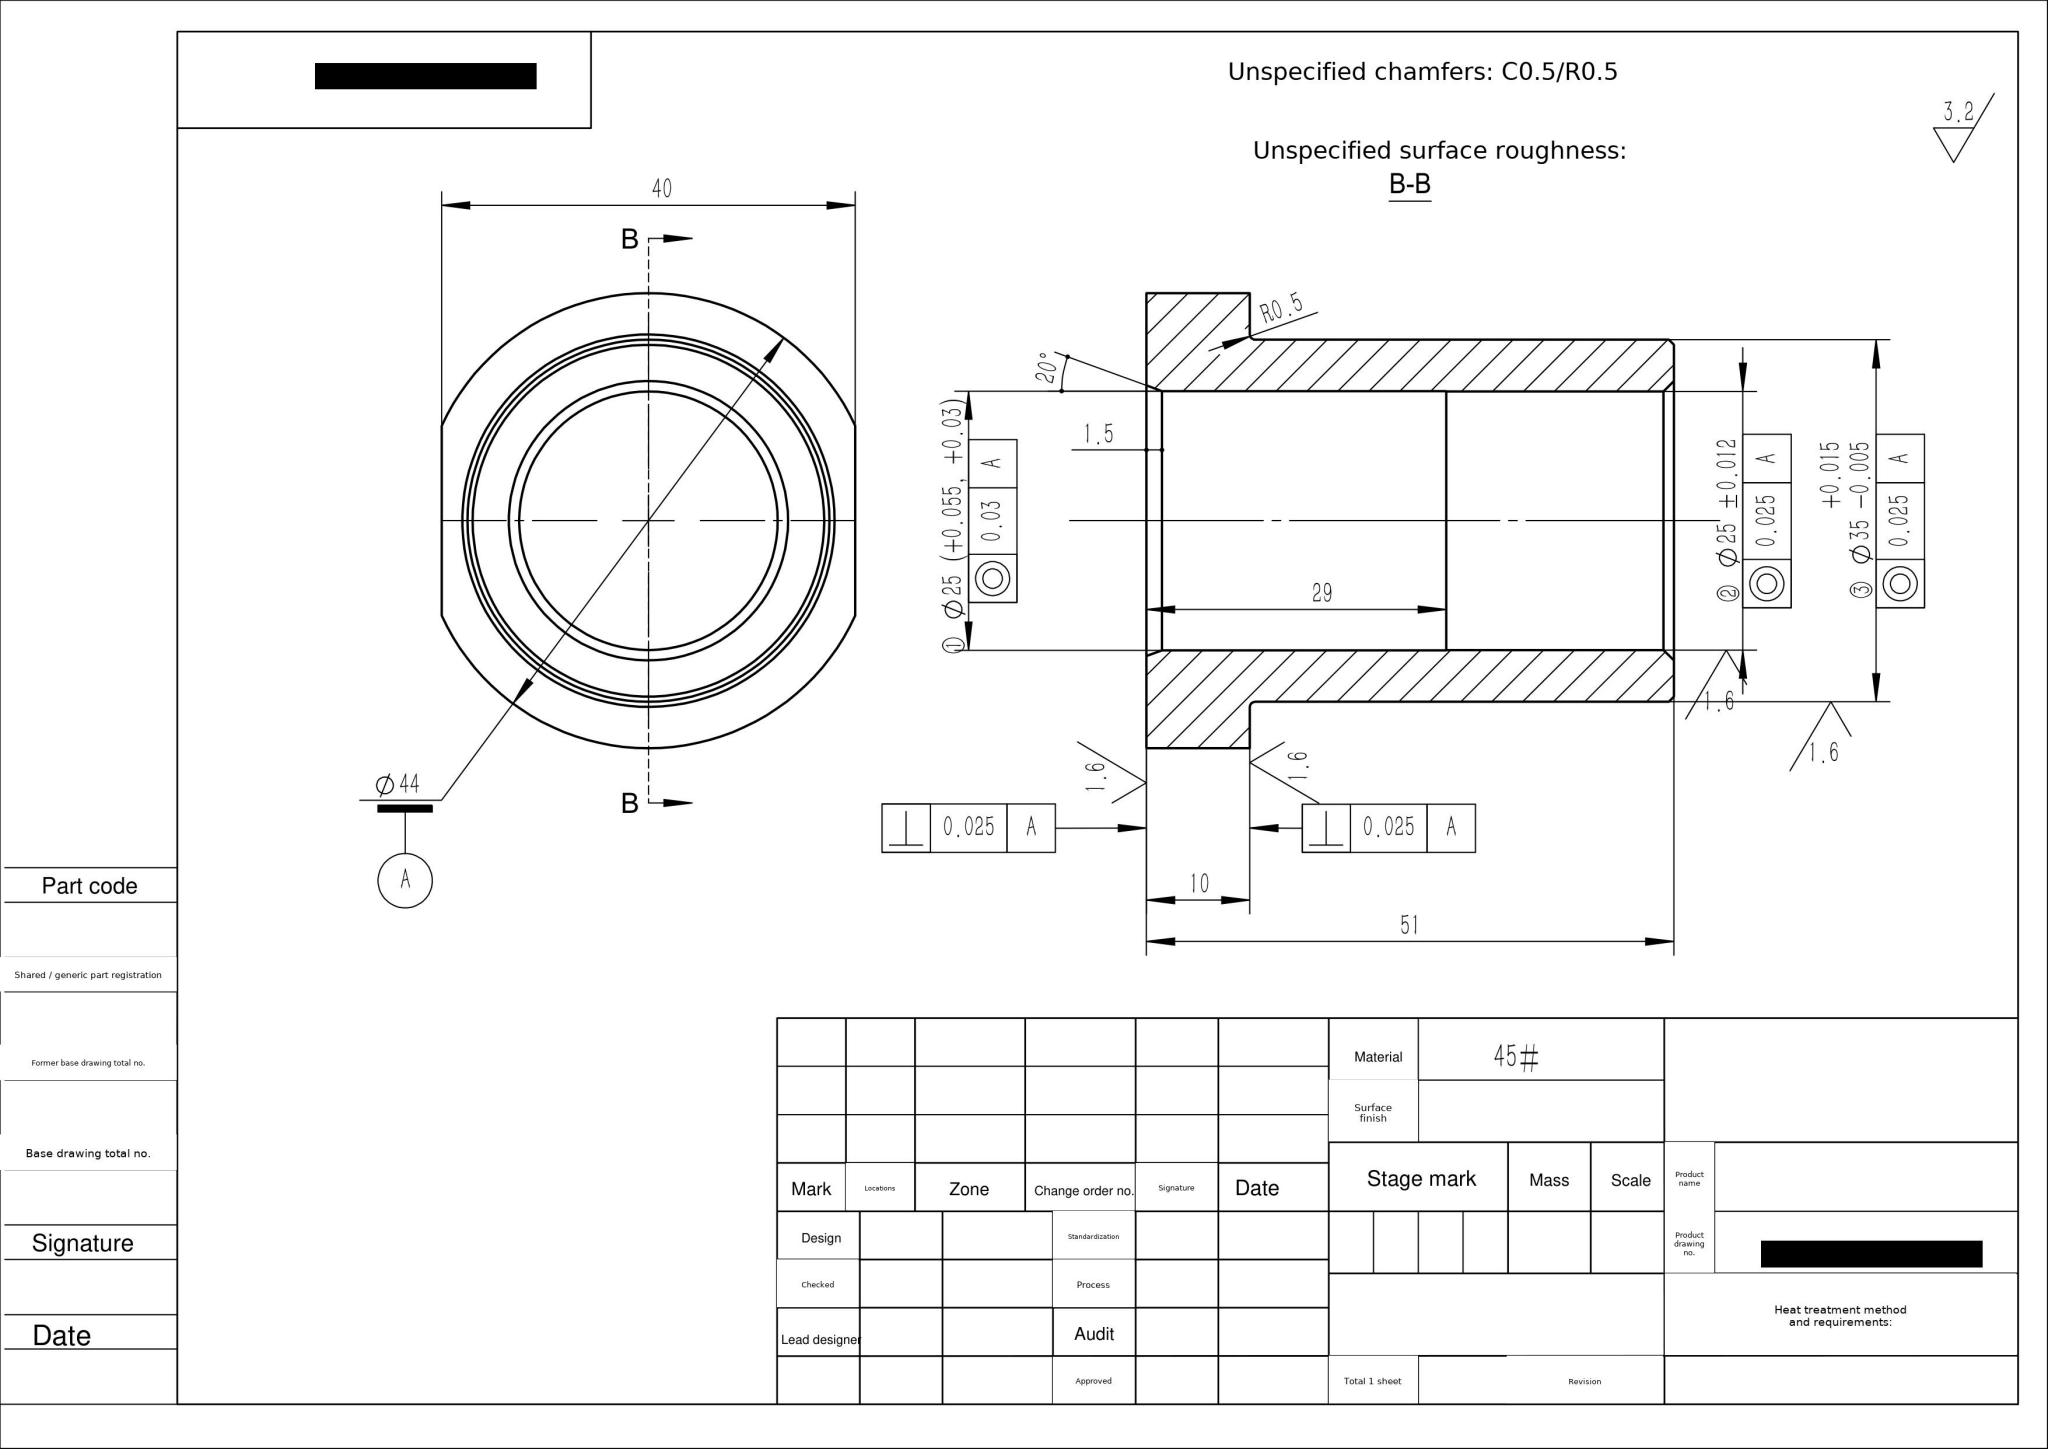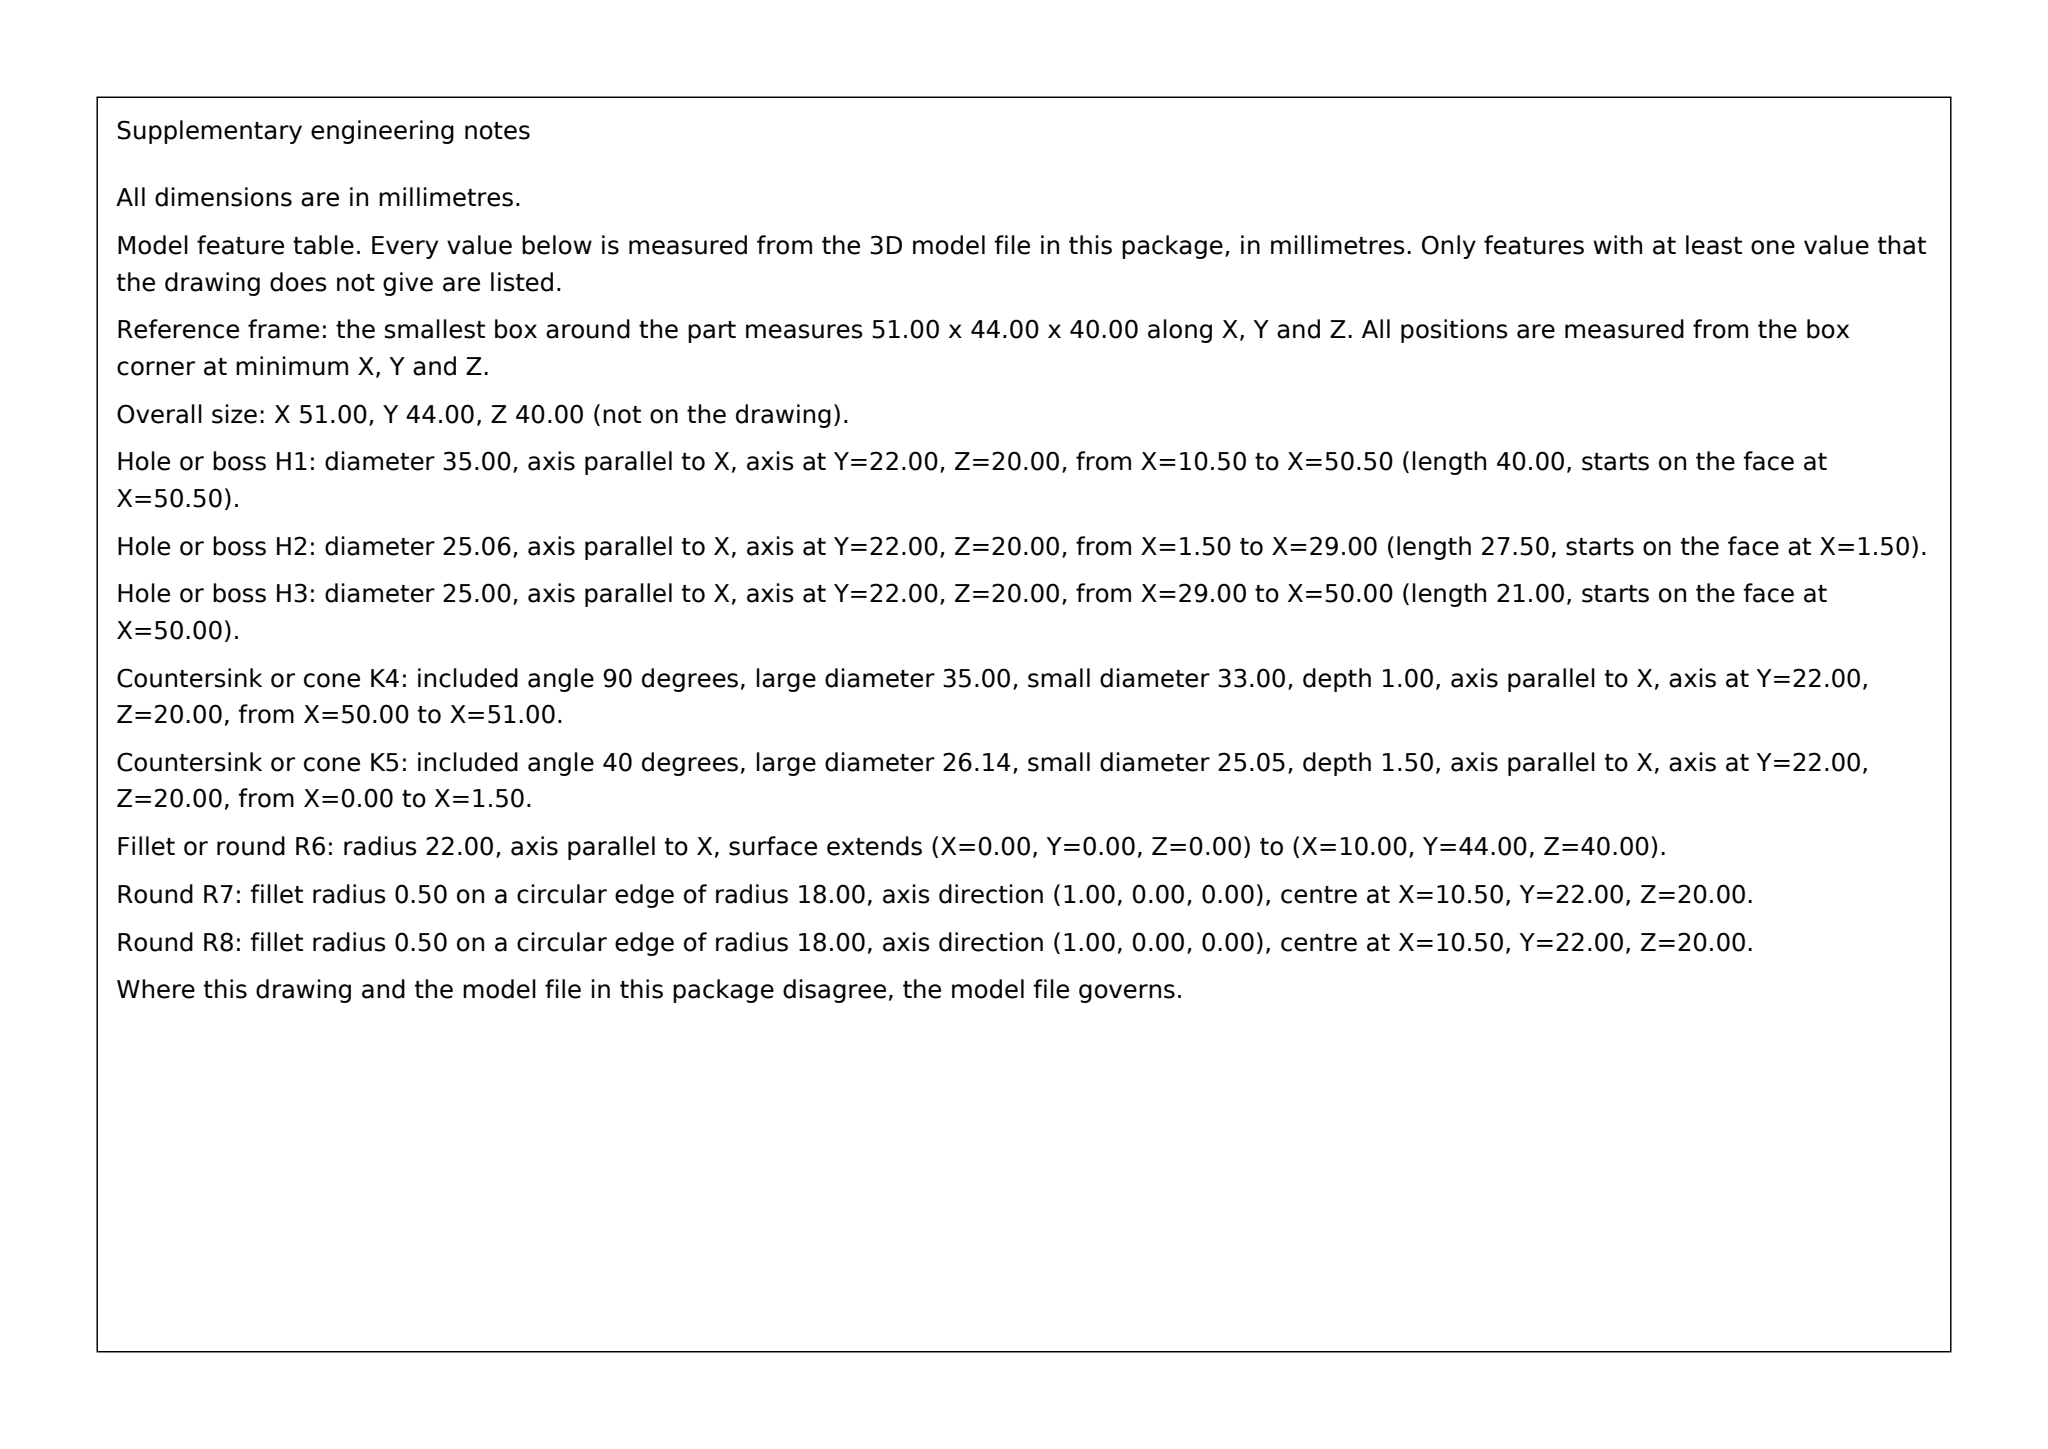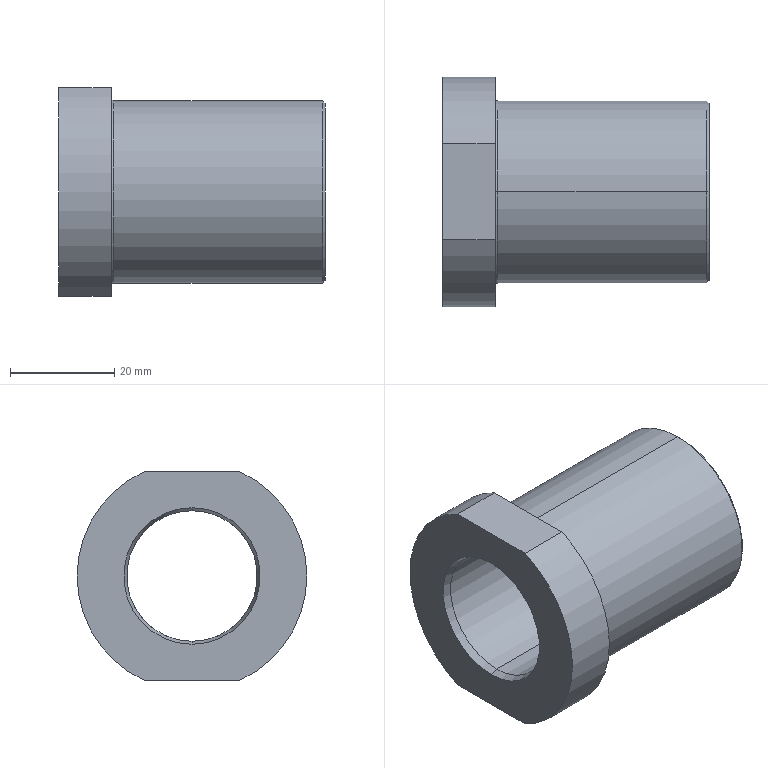Part | SolidWorks | mm | material 45# | 1 solid | 22 faces | box 51 x 44 x 40 mm | volume 28986 mm3 | cylinder 8 | cone 6 | plane 6 | torus 2 | commonest cylinder face diameters 25 x2 35 x2 25.05 x2 44 x2
STEP:
#1=CARTESIAN_POINT('',(50.,0.,12.5));
#2=VERTEX_POINT('',#1);
#3=CARTESIAN_POINT('',(50.,0.,-12.5));
#4=VERTEX_POINT('',#3);
#5=CARTESIAN_POINT('',(50.,0.,0.));
#6=DIRECTION('',(1.,0.,0.));
#7=DIRECTION('',(0.,0.,-1.));
#8=AXIS2_PLACEMENT_3D('',#5,#6,#7);
#9=CIRCLE('',#8,12.5);
#10=EDGE_CURVE('',#2,#4,#9,.T.);
#11=ORIENTED_EDGE('',*,*,#10,.F.);
#12=CARTESIAN_POINT('',(51.,0.,13.5));
#13=VERTEX_POINT('',#12);
#14=CARTESIAN_POINT('',(50.,0.,12.5));
#15=DIRECTION('',(0.7071,0.,0.7071));
#16=VECTOR('',#15,1000.);
#17=LINE('',#14,#16);
#18=EDGE_CURVE('',#2,#13,#17,.T.);
#19=ORIENTED_EDGE('',*,*,#18,.T.);
#20=CARTESIAN_POINT('',(51.,0.,-13.5));
#21=VERTEX_POINT('',#20);
#22=CARTESIAN_POINT('',(51.,0.,0.));
#23=DIRECTION('',(-1.,0.,0.));
#24=DIRECTION('',(0.,0.,-1.));
#25=AXIS2_PLACEMENT_3D('',#22,#23,#24);
#26=CIRCLE('',#25,13.5);
#27=EDGE_CURVE('',#21,#13,#26,.T.);
#28=ORIENTED_EDGE('',*,*,#27,.F.);
#29=CARTESIAN_POINT('',(50.,0.,-12.5));
#30=DIRECTION('',(0.7071,0.,-0.7071));
#31=VECTOR('',#30,1000.);
#32=LINE('',#29,#31);
#33=EDGE_CURVE('',#4,#21,#32,.T.);
#34=ORIENTED_EDGE('',*,*,#33,.F.);
#35=EDGE_LOOP('',(#11,#19,#28,#34));
#36=FACE_OUTER_BOUND('',#35,.T.);
#37=CARTESIAN_POINT('',(50.,0.,0.));
#38=DIRECTION('',(1.,0.,0.));
#39=DIRECTION('',(0.,0.,-1.));
#40=AXIS2_PLACEMENT_3D('',#37,#38,#39);
#41=CONICAL_SURFACE('',#40,12.5,0.7854);
#42=ADVANCED_FACE('',(#36),#41,.F.);
#43=CARTESIAN_POINT('',(29.,0.,12.5));
#44=VERTEX_POINT('',#43);
#45=CARTESIAN_POINT('',(29.,0.,-12.5));
#46=VERTEX_POINT('',#45);
#47=CARTESIAN_POINT('',(29.,0.,0.));
#48=DIRECTION('',(1.,0.,0.));
#49=DIRECTION('',(0.,0.,-1.));
#50=AXIS2_PLACEMENT_3D('',#47,#48,#49);
#51=CIRCLE('',#50,12.5);
#52=EDGE_CURVE('',#44,#46,#51,.T.);
#53=ORIENTED_EDGE('',*,*,#52,.F.);
#54=CARTESIAN_POINT('',(29.,0.,12.5));
#55=DIRECTION('',(1.,0.,0.));
#56=VECTOR('',#55,1000.);
#57=LINE('',#54,#56);
#58=EDGE_CURVE('',#44,#2,#57,.T.);
#59=ORIENTED_EDGE('',*,*,#58,.T.);
#60=ORIENTED_EDGE('',*,*,#10,.T.);
#61=CARTESIAN_POINT('',(29.,0.,-12.5));
#62=DIRECTION('',(1.,0.,0.));
#63=VECTOR('',#62,1000.);
#64=LINE('',#61,#63);
#65=EDGE_CURVE('',#46,#4,#64,.T.);
#66=ORIENTED_EDGE('',*,*,#65,.F.);
#67=EDGE_LOOP('',(#53,#59,#60,#66));
#68=FACE_OUTER_BOUND('',#67,.T.);
#69=CARTESIAN_POINT('',(29.,0.,0.));
#70=DIRECTION('',(1.,0.,0.));
#71=DIRECTION('',(0.,0.,-1.));
#72=AXIS2_PLACEMENT_3D('',#69,#70,#71);
#73=CYLINDRICAL_SURFACE('',#72,12.5);
#74=ADVANCED_FACE('',(#68),#73,.F.);
#75=CARTESIAN_POINT('',(1.5,0.,-12.525));
#76=VERTEX_POINT('',#75);
#77=CARTESIAN_POINT('',(1.5,0.,12.525));
#78=VERTEX_POINT('',#77);
#79=CARTESIAN_POINT('',(1.5,0.,0.));
#80=DIRECTION('',(-1.,0.,0.));
#81=DIRECTION('',(0.,0.,-1.));
#82=AXIS2_PLACEMENT_3D('',#79,#80,#81);
#83=CIRCLE('',#82,12.525);
#84=EDGE_CURVE('',#76,#78,#83,.T.);
#85=ORIENTED_EDGE('',*,*,#84,.F.);
#86=CARTESIAN_POINT('',(0.,0.,-13.071));
#87=VERTEX_POINT('',#86);
#88=CARTESIAN_POINT('',(1.5,0.,-12.525));
#89=DIRECTION('',(-0.9397,0.,-0.342));
#90=VECTOR('',#89,1000.);
#91=LINE('',#88,#90);
#92=EDGE_CURVE('',#76,#87,#91,.T.);
#93=ORIENTED_EDGE('',*,*,#92,.T.);
#94=CARTESIAN_POINT('',(0.,0.,13.071));
#95=VERTEX_POINT('',#94);
#96=CARTESIAN_POINT('',(0.,0.,0.));
#97=DIRECTION('',(1.,0.,0.));
#98=DIRECTION('',(0.,0.,-1.));
#99=AXIS2_PLACEMENT_3D('',#96,#97,#98);
#100=CIRCLE('',#99,13.071);
#101=EDGE_CURVE('',#95,#87,#100,.T.);
#102=ORIENTED_EDGE('',*,*,#101,.F.);
#103=CARTESIAN_POINT('',(1.5,0.,12.525));
#104=DIRECTION('',(-0.9397,0.,0.342));
#105=VECTOR('',#104,1000.);
#106=LINE('',#103,#105);
#107=EDGE_CURVE('',#78,#95,#106,.T.);
#108=ORIENTED_EDGE('',*,*,#107,.F.);
#109=EDGE_LOOP('',(#85,#93,#102,#108));
#110=FACE_OUTER_BOUND('',#109,.T.);
#111=CARTESIAN_POINT('',(1.5,0.,0.));
#112=DIRECTION('',(-1.,0.,0.));
#113=DIRECTION('',(0.,0.,1.));
#114=AXIS2_PLACEMENT_3D('',#111,#112,#113);
#115=CONICAL_SURFACE('',#114,12.525,0.3491);
#116=ADVANCED_FACE('',(#110),#115,.F.);
#117=CARTESIAN_POINT('',(51.,0.,-17.));
#118=VERTEX_POINT('',#117);
#119=CARTESIAN_POINT('',(51.,0.,17.));
#120=VERTEX_POINT('',#119);
#121=CARTESIAN_POINT('',(51.,0.,0.));
#122=DIRECTION('',(1.,0.,0.));
#123=DIRECTION('',(0.,0.,-1.));
#124=AXIS2_PLACEMENT_3D('',#121,#122,#123);
#125=CIRCLE('',#124,17.);
#126=EDGE_CURVE('',#118,#120,#125,.T.);
#127=ORIENTED_EDGE('',*,*,#126,.F.);
#128=CARTESIAN_POINT('',(50.5,0.,-17.5));
#129=VERTEX_POINT('',#128);
#130=CARTESIAN_POINT('',(51.,0.,-17.));
#131=DIRECTION('',(-0.7071,0.,-0.7071));
#132=VECTOR('',#131,1000.);
#133=LINE('',#130,#132);
#134=EDGE_CURVE('',#118,#129,#133,.T.);
#135=ORIENTED_EDGE('',*,*,#134,.T.);
#136=CARTESIAN_POINT('',(50.5,0.,17.5));
#137=VERTEX_POINT('',#136);
#138=CARTESIAN_POINT('',(50.5,0.,0.));
#139=DIRECTION('',(-1.,0.,0.));
#140=DIRECTION('',(0.,0.,-1.));
#141=AXIS2_PLACEMENT_3D('',#138,#139,#140);
#142=CIRCLE('',#141,17.5);
#143=EDGE_CURVE('',#137,#129,#142,.T.);
#144=ORIENTED_EDGE('',*,*,#143,.F.);
#145=CARTESIAN_POINT('',(51.,0.,17.));
#146=DIRECTION('',(-0.7071,0.,0.7071));
#147=VECTOR('',#146,1000.);
#148=LINE('',#145,#147);
#149=EDGE_CURVE('',#120,#137,#148,.T.);
#150=ORIENTED_EDGE('',*,*,#149,.F.);
#151=EDGE_LOOP('',(#127,#135,#144,#150));
#152=FACE_OUTER_BOUND('',#151,.T.);
#153=CARTESIAN_POINT('',(51.,0.,0.));
#154=DIRECTION('',(-1.,0.,0.));
#155=DIRECTION('',(0.,0.,1.));
#156=AXIS2_PLACEMENT_3D('',#153,#154,#155);
#157=CONICAL_SURFACE('',#156,17.,0.7854);
#158=ADVANCED_FACE('',(#152),#157,.T.);
#159=CARTESIAN_POINT('',(10.5,0.,17.5));
#160=VERTEX_POINT('',#159);
#161=CARTESIAN_POINT('',(10.5,0.,-17.5));
#162=VERTEX_POINT('',#161);
#163=CARTESIAN_POINT('',(10.5,0.,0.));
#164=DIRECTION('',(1.,0.,0.));
#165=DIRECTION('',(0.,0.,-1.));
#166=AXIS2_PLACEMENT_3D('',#163,#164,#165);
#167=CIRCLE('',#166,17.5);
#168=EDGE_CURVE('',#160,#162,#167,.T.);
#169=ORIENTED_EDGE('',*,*,#168,.F.);
#170=CARTESIAN_POINT('',(10.,0.,18.));
#171=VERTEX_POINT('',#170);
#172=CARTESIAN_POINT('',(10.5,0.,18.));
#173=DIRECTION('',(0.,1.,-0.));
#174=DIRECTION('',(0.,0.,1.));
#175=AXIS2_PLACEMENT_3D('',#172,#173,#174);
#176=CIRCLE('',#175,0.5);
#177=EDGE_CURVE('',#160,#171,#176,.T.);
#178=ORIENTED_EDGE('',*,*,#177,.T.);
#179=CARTESIAN_POINT('',(10.,0.,-18.));
#180=VERTEX_POINT('',#179);
#181=CARTESIAN_POINT('',(10.,0.,0.));
#182=DIRECTION('',(-1.,0.,0.));
#183=DIRECTION('',(0.,0.,-1.));
#184=AXIS2_PLACEMENT_3D('',#181,#182,#183);
#185=CIRCLE('',#184,18.);
#186=EDGE_CURVE('',#180,#171,#185,.T.);
#187=ORIENTED_EDGE('',*,*,#186,.F.);
#188=CARTESIAN_POINT('',(10.5,0.,-18.));
#189=DIRECTION('',(0.,-1.,0.));
#190=DIRECTION('',(0.,0.,-1.));
#191=AXIS2_PLACEMENT_3D('',#188,#189,#190);
#192=CIRCLE('',#191,0.5);
#193=EDGE_CURVE('',#162,#180,#192,.T.);
#194=ORIENTED_EDGE('',*,*,#193,.F.);
#195=EDGE_LOOP('',(#169,#178,#187,#194));
#196=FACE_OUTER_BOUND('',#195,.T.);
#197=CARTESIAN_POINT('',(10.5,0.,0.));
#198=DIRECTION('',(1.,0.,0.));
#199=DIRECTION('',(0.,0.,-1.));
#200=AXIS2_PLACEMENT_3D('',#197,#198,#199);
#201=TOROIDAL_SURFACE('',#200,18.,0.5);
#202=ADVANCED_FACE('',(#196),#201,.F.);
#203=ORIENTED_EDGE('',*,*,#143,.T.);
#204=CARTESIAN_POINT('',(51.,0.,-17.5));
#205=DIRECTION('',(-1.,0.,0.));
#206=VECTOR('',#205,1000.);
#207=LINE('',#204,#206);
#208=EDGE_CURVE('',#129,#162,#207,.T.);
#209=ORIENTED_EDGE('',*,*,#208,.T.);
#210=CARTESIAN_POINT('',(10.5,0.,0.));
#211=DIRECTION('',(1.,0.,0.));
#212=DIRECTION('',(0.,0.,-1.));
#213=AXIS2_PLACEMENT_3D('',#210,#211,#212);
#214=CIRCLE('',#213,17.5);
#215=EDGE_CURVE('',#162,#160,#214,.T.);
#216=ORIENTED_EDGE('',*,*,#215,.T.);
#217=CARTESIAN_POINT('',(51.,0.,17.5));
#218=DIRECTION('',(-1.,0.,0.));
#219=VECTOR('',#218,1000.);
#220=LINE('',#217,#219);
#221=EDGE_CURVE('',#137,#160,#220,.T.);
#222=ORIENTED_EDGE('',*,*,#221,.F.);
#223=EDGE_LOOP('',(#203,#209,#216,#222));
#224=FACE_OUTER_BOUND('',#223,.T.);
#225=CARTESIAN_POINT('',(51.,0.,0.));
#226=DIRECTION('',(-1.,0.,0.));
#227=DIRECTION('',(0.,0.,1.));
#228=AXIS2_PLACEMENT_3D('',#225,#226,#227);
#229=CYLINDRICAL_SURFACE('',#228,17.5);
#230=ADVANCED_FACE('',(#224),#229,.T.);
#231=CARTESIAN_POINT('',(29.,0.,-12.525));
#232=VERTEX_POINT('',#231);
#233=CARTESIAN_POINT('',(29.,0.,12.525));
#234=VERTEX_POINT('',#233);
#235=CARTESIAN_POINT('',(29.,0.,0.));
#236=DIRECTION('',(-1.,0.,0.));
#237=DIRECTION('',(0.,0.,-1.));
#238=AXIS2_PLACEMENT_3D('',#235,#236,#237);
#239=CIRCLE('',#238,12.525);
#240=EDGE_CURVE('',#232,#234,#239,.T.);
#241=ORIENTED_EDGE('',*,*,#240,.F.);
#242=CARTESIAN_POINT('',(51.,0.,-12.525));
#243=DIRECTION('',(-1.,0.,0.));
#244=VECTOR('',#243,1000.);
#245=LINE('',#242,#244);
#246=EDGE_CURVE('',#232,#76,#245,.T.);
#247=ORIENTED_EDGE('',*,*,#246,.T.);
#248=ORIENTED_EDGE('',*,*,#84,.T.);
#249=CARTESIAN_POINT('',(51.,0.,12.525));
#250=DIRECTION('',(-1.,0.,0.));
#251=VECTOR('',#250,1000.);
#252=LINE('',#249,#251);
#253=EDGE_CURVE('',#234,#78,#252,.T.);
#254=ORIENTED_EDGE('',*,*,#253,.F.);
#255=EDGE_LOOP('',(#241,#247,#248,#254));
#256=FACE_OUTER_BOUND('',#255,.T.);
#257=CARTESIAN_POINT('',(51.,0.,0.));
#258=DIRECTION('',(-1.,0.,0.));
#259=DIRECTION('',(0.,0.,1.));
#260=AXIS2_PLACEMENT_3D('',#257,#258,#259);
#261=CYLINDRICAL_SURFACE('',#260,12.525);
#262=ADVANCED_FACE('',(#256),#261,.F.);
#263=ORIENTED_EDGE('',*,*,#246,.F.);
#264=CARTESIAN_POINT('',(29.,0.,0.));
#265=DIRECTION('',(-1.,0.,0.));
#266=DIRECTION('',(0.,0.,-1.));
#267=AXIS2_PLACEMENT_3D('',#264,#265,#266);
#268=CIRCLE('',#267,12.525);
#269=EDGE_CURVE('',#234,#232,#268,.T.);
#270=ORIENTED_EDGE('',*,*,#269,.F.);
#271=ORIENTED_EDGE('',*,*,#253,.T.);
#272=CARTESIAN_POINT('',(1.5,0.,0.));
#273=DIRECTION('',(-1.,0.,0.));
#274=DIRECTION('',(0.,0.,-1.));
#275=AXIS2_PLACEMENT_3D('',#272,#273,#274);
#276=CIRCLE('',#275,12.525);
#277=EDGE_CURVE('',#78,#76,#276,.T.);
#278=ORIENTED_EDGE('',*,*,#277,.T.);
#279=EDGE_LOOP('',(#263,#270,#271,#278));
#280=FACE_OUTER_BOUND('',#279,.T.);
#281=CARTESIAN_POINT('',(51.,0.,0.));
#282=DIRECTION('',(-1.,0.,0.));
#283=DIRECTION('',(0.,0.,1.));
#284=AXIS2_PLACEMENT_3D('',#281,#282,#283);
#285=CYLINDRICAL_SURFACE('',#284,12.525);
#286=ADVANCED_FACE('',(#280),#285,.F.);
#287=CARTESIAN_POINT('',(10.,9.165,20.));
#288=VERTEX_POINT('',#287);
#289=CARTESIAN_POINT('',(0.,9.165,20.));
#290=VERTEX_POINT('',#289);
#291=CARTESIAN_POINT('',(10.,9.165,20.));
#292=DIRECTION('',(-1.,0.,0.));
#293=VECTOR('',#292,1000.);
#294=LINE('',#291,#293);
#295=EDGE_CURVE('',#288,#290,#294,.T.);
#296=ORIENTED_EDGE('',*,*,#295,.F.);
#297=CARTESIAN_POINT('',(10.,9.165,-20.));
#298=VERTEX_POINT('',#297);
#299=CARTESIAN_POINT('',(10.,0.,0.));
#300=DIRECTION('',(1.,0.,0.));
#301=DIRECTION('',(0.,0.,-1.));
#302=AXIS2_PLACEMENT_3D('',#299,#300,#301);
#303=CIRCLE('',#302,22.);
#304=EDGE_CURVE('',#298,#288,#303,.T.);
#305=ORIENTED_EDGE('',*,*,#304,.F.);
#306=CARTESIAN_POINT('',(0.,9.165,-20.));
#307=VERTEX_POINT('',#306);
#308=CARTESIAN_POINT('',(10.,9.165,-20.));
#309=DIRECTION('',(1.,0.,0.));
#310=VECTOR('',#309,1000.);
#311=LINE('',#308,#310);
#312=EDGE_CURVE('',#307,#298,#311,.T.);
#313=ORIENTED_EDGE('',*,*,#312,.F.);
#314=CARTESIAN_POINT('',(0.,0.,0.));
#315=DIRECTION('',(1.,0.,0.));
#316=DIRECTION('',(0.,0.,-1.));
#317=AXIS2_PLACEMENT_3D('',#314,#315,#316);
#318=CIRCLE('',#317,22.);
#319=EDGE_CURVE('',#307,#290,#318,.T.);
#320=ORIENTED_EDGE('',*,*,#319,.T.);
#321=EDGE_LOOP('',(#296,#305,#313,#320));
#322=FACE_OUTER_BOUND('',#321,.T.);
#323=CARTESIAN_POINT('',(10.,0.,0.));
#324=DIRECTION('',(-1.,0.,0.));
#325=DIRECTION('',(0.,0.,1.));
#326=AXIS2_PLACEMENT_3D('',#323,#324,#325);
#327=CYLINDRICAL_SURFACE('',#326,22.);
#328=ADVANCED_FACE('',(#322),#327,.T.);
#329=CARTESIAN_POINT('',(0.,-9.165,20.));
#330=VERTEX_POINT('',#329);
#331=CARTESIAN_POINT('',(10.,-9.165,20.));
#332=VERTEX_POINT('',#331);
#333=CARTESIAN_POINT('',(10.,-9.165,20.));
#334=DIRECTION('',(1.,0.,0.));
#335=VECTOR('',#334,1000.);
#336=LINE('',#333,#335);
#337=EDGE_CURVE('',#330,#332,#336,.T.);
#338=ORIENTED_EDGE('',*,*,#337,.F.);
#339=CARTESIAN_POINT('',(0.,-9.165,-20.));
#340=VERTEX_POINT('',#339);
#341=CARTESIAN_POINT('',(0.,0.,0.));
#342=DIRECTION('',(1.,0.,0.));
#343=DIRECTION('',(0.,0.,-1.));
#344=AXIS2_PLACEMENT_3D('',#341,#342,#343);
#345=CIRCLE('',#344,22.);
#346=EDGE_CURVE('',#330,#340,#345,.T.);
#347=ORIENTED_EDGE('',*,*,#346,.T.);
#348=CARTESIAN_POINT('',(10.,-9.165,-20.));
#349=VERTEX_POINT('',#348);
#350=CARTESIAN_POINT('',(10.,-9.165,-20.));
#351=DIRECTION('',(-1.,0.,0.));
#352=VECTOR('',#351,1000.);
#353=LINE('',#350,#352);
#354=EDGE_CURVE('',#349,#340,#353,.T.);
#355=ORIENTED_EDGE('',*,*,#354,.F.);
#356=CARTESIAN_POINT('',(10.,0.,0.));
#357=DIRECTION('',(1.,0.,0.));
#358=DIRECTION('',(0.,0.,-1.));
#359=AXIS2_PLACEMENT_3D('',#356,#357,#358);
#360=CIRCLE('',#359,22.);
#361=EDGE_CURVE('',#332,#349,#360,.T.);
#362=ORIENTED_EDGE('',*,*,#361,.F.);
#363=EDGE_LOOP('',(#338,#347,#355,#362));
#364=FACE_OUTER_BOUND('',#363,.T.);
#365=CARTESIAN_POINT('',(10.,0.,0.));
#366=DIRECTION('',(-1.,0.,0.));
#367=DIRECTION('',(0.,0.,1.));
#368=AXIS2_PLACEMENT_3D('',#365,#366,#367);
#369=CYLINDRICAL_SURFACE('',#368,22.);
#370=ADVANCED_FACE('',(#364),#369,.T.);
#371=ORIENTED_EDGE('',*,*,#186,.T.);
#372=CARTESIAN_POINT('',(10.,0.,0.));
#373=DIRECTION('',(-1.,0.,0.));
#374=DIRECTION('',(0.,0.,-1.));
#375=AXIS2_PLACEMENT_3D('',#372,#373,#374);
#376=CIRCLE('',#375,18.);
#377=EDGE_CURVE('',#171,#180,#376,.T.);
#378=ORIENTED_EDGE('',*,*,#377,.T.);
#379=EDGE_LOOP('',(#371,#378));
#380=FACE_BOUND('',#379,.T.);
#381=ORIENTED_EDGE('',*,*,#304,.T.);
#382=CARTESIAN_POINT('',(10.,0.,20.));
#383=DIRECTION('',(0.,-1.,0.));
#384=VECTOR('',#383,1000.);
#385=LINE('',#382,#384);
#386=EDGE_CURVE('',#288,#332,#385,.T.);
#387=ORIENTED_EDGE('',*,*,#386,.T.);
#388=ORIENTED_EDGE('',*,*,#361,.T.);
#389=CARTESIAN_POINT('',(10.,-0.,-20.));
#390=DIRECTION('',(0.,1.,-0.));
#391=VECTOR('',#390,1000.);
#392=LINE('',#389,#391);
#393=EDGE_CURVE('',#349,#298,#392,.T.);
#394=ORIENTED_EDGE('',*,*,#393,.T.);
#395=EDGE_LOOP('',(#381,#387,#388,#394));
#396=FACE_OUTER_BOUND('',#395,.T.);
#397=CARTESIAN_POINT('',(10.,0.,0.));
#398=DIRECTION('',(1.,0.,0.));
#399=DIRECTION('',(0.,0.,-1.));
#400=AXIS2_PLACEMENT_3D('',#397,#398,#399);
#401=PLANE('',#400);
#402=ADVANCED_FACE('',(#380,#396),#401,.T.);
#403=ORIENTED_EDGE('',*,*,#101,.T.);
#404=CARTESIAN_POINT('',(0.,0.,0.));
#405=DIRECTION('',(1.,0.,0.));
#406=DIRECTION('',(0.,0.,-1.));
#407=AXIS2_PLACEMENT_3D('',#404,#405,#406);
#408=CIRCLE('',#407,13.071);
#409=EDGE_CURVE('',#87,#95,#408,.T.);
#410=ORIENTED_EDGE('',*,*,#409,.T.);
#411=EDGE_LOOP('',(#403,#410));
#412=FACE_BOUND('',#411,.T.);
#413=CARTESIAN_POINT('',(0.,0.,20.));
#414=DIRECTION('',(0.,-1.,0.));
#415=VECTOR('',#414,1000.);
#416=LINE('',#413,#415);
#417=EDGE_CURVE('',#290,#330,#416,.T.);
#418=ORIENTED_EDGE('',*,*,#417,.F.);
#419=ORIENTED_EDGE('',*,*,#319,.F.);
#420=CARTESIAN_POINT('',(0.,-0.,-20.));
#421=DIRECTION('',(0.,1.,-0.));
#422=VECTOR('',#421,1000.);
#423=LINE('',#420,#422);
#424=EDGE_CURVE('',#340,#307,#423,.T.);
#425=ORIENTED_EDGE('',*,*,#424,.F.);
#426=ORIENTED_EDGE('',*,*,#346,.F.);
#427=EDGE_LOOP('',(#418,#419,#425,#426));
#428=FACE_OUTER_BOUND('',#427,.T.);
#429=CARTESIAN_POINT('',(0.,0.,0.));
#430=DIRECTION('',(1.,0.,0.));
#431=DIRECTION('',(0.,0.,-1.));
#432=AXIS2_PLACEMENT_3D('',#429,#430,#431);
#433=PLANE('',#432);
#434=ADVANCED_FACE('',(#412,#428),#433,.F.);
#435=ORIENTED_EDGE('',*,*,#208,.F.);
#436=CARTESIAN_POINT('',(50.5,0.,0.));
#437=DIRECTION('',(-1.,0.,0.));
#438=DIRECTION('',(0.,0.,-1.));
#439=AXIS2_PLACEMENT_3D('',#436,#437,#438);
#440=CIRCLE('',#439,17.5);
#441=EDGE_CURVE('',#129,#137,#440,.T.);
#442=ORIENTED_EDGE('',*,*,#441,.T.);
#443=ORIENTED_EDGE('',*,*,#221,.T.);
#444=ORIENTED_EDGE('',*,*,#168,.T.);
#445=EDGE_LOOP('',(#435,#442,#443,#444));
#446=FACE_OUTER_BOUND('',#445,.T.);
#447=CARTESIAN_POINT('',(51.,0.,0.));
#448=DIRECTION('',(-1.,0.,0.));
#449=DIRECTION('',(0.,0.,1.));
#450=AXIS2_PLACEMENT_3D('',#447,#448,#449);
#451=CYLINDRICAL_SURFACE('',#450,17.5);
#452=ADVANCED_FACE('',(#446),#451,.T.);
#453=ORIENTED_EDGE('',*,*,#27,.T.);
#454=CARTESIAN_POINT('',(51.,0.,0.));
#455=DIRECTION('',(-1.,0.,0.));
#456=DIRECTION('',(0.,0.,-1.));
#457=AXIS2_PLACEMENT_3D('',#454,#455,#456);
#458=CIRCLE('',#457,13.5);
#459=EDGE_CURVE('',#13,#21,#458,.T.);
#460=ORIENTED_EDGE('',*,*,#459,.T.);
#461=EDGE_LOOP('',(#453,#460));
#462=FACE_BOUND('',#461,.T.);
#463=CARTESIAN_POINT('',(51.,0.,0.));
#464=DIRECTION('',(1.,0.,0.));
#465=DIRECTION('',(0.,0.,-1.));
#466=AXIS2_PLACEMENT_3D('',#463,#464,#465);
#467=CIRCLE('',#466,17.);
#468=EDGE_CURVE('',#120,#118,#467,.T.);
#469=ORIENTED_EDGE('',*,*,#468,.T.);
#470=ORIENTED_EDGE('',*,*,#126,.T.);
#471=EDGE_LOOP('',(#469,#470));
#472=FACE_OUTER_BOUND('',#471,.T.);
#473=CARTESIAN_POINT('',(51.,0.,0.));
#474=DIRECTION('',(1.,0.,0.));
#475=DIRECTION('',(0.,0.,-1.));
#476=AXIS2_PLACEMENT_3D('',#473,#474,#475);
#477=PLANE('',#476);
#478=ADVANCED_FACE('',(#462,#472),#477,.T.);
#479=ORIENTED_EDGE('',*,*,#354,.T.);
#480=ORIENTED_EDGE('',*,*,#424,.T.);
#481=ORIENTED_EDGE('',*,*,#312,.T.);
#482=ORIENTED_EDGE('',*,*,#393,.F.);
#483=EDGE_LOOP('',(#479,#480,#481,#482));
#484=FACE_OUTER_BOUND('',#483,.T.);
#485=CARTESIAN_POINT('',(51.,31.237,-20.));
#486=DIRECTION('',(0.,-0.,-1.));
#487=DIRECTION('',(0.,1.,-0.));
#488=AXIS2_PLACEMENT_3D('',#485,#486,#487);
#489=PLANE('',#488);
#490=ADVANCED_FACE('',(#484),#489,.T.);
#491=ORIENTED_EDGE('',*,*,#295,.T.);
#492=ORIENTED_EDGE('',*,*,#417,.T.);
#493=ORIENTED_EDGE('',*,*,#337,.T.);
#494=ORIENTED_EDGE('',*,*,#386,.F.);
#495=EDGE_LOOP('',(#491,#492,#493,#494));
#496=FACE_OUTER_BOUND('',#495,.T.);
#497=CARTESIAN_POINT('',(51.,31.237,20.));
#498=DIRECTION('',(0.,0.,1.));
#499=DIRECTION('',(0.,-1.,0.));
#500=AXIS2_PLACEMENT_3D('',#497,#498,#499);
#501=PLANE('',#500);
#502=ADVANCED_FACE('',(#496),#501,.T.);
#503=ORIENTED_EDGE('',*,*,#177,.F.);
#504=ORIENTED_EDGE('',*,*,#215,.F.);
#505=ORIENTED_EDGE('',*,*,#193,.T.);
#506=ORIENTED_EDGE('',*,*,#377,.F.);
#507=EDGE_LOOP('',(#503,#504,#505,#506));
#508=FACE_OUTER_BOUND('',#507,.T.);
#509=CARTESIAN_POINT('',(10.5,0.,0.));
#510=DIRECTION('',(1.,0.,0.));
#511=DIRECTION('',(0.,0.,-1.));
#512=AXIS2_PLACEMENT_3D('',#509,#510,#511);
#513=TOROIDAL_SURFACE('',#512,18.,0.5);
#514=ADVANCED_FACE('',(#508),#513,.F.);
#515=ORIENTED_EDGE('',*,*,#134,.F.);
#516=ORIENTED_EDGE('',*,*,#468,.F.);
#517=ORIENTED_EDGE('',*,*,#149,.T.);
#518=ORIENTED_EDGE('',*,*,#441,.F.);
#519=EDGE_LOOP('',(#515,#516,#517,#518));
#520=FACE_OUTER_BOUND('',#519,.T.);
#521=CARTESIAN_POINT('',(51.,0.,0.));
#522=DIRECTION('',(-1.,0.,0.));
#523=DIRECTION('',(0.,0.,1.));
#524=AXIS2_PLACEMENT_3D('',#521,#522,#523);
#525=CONICAL_SURFACE('',#524,17.,0.7854);
#526=ADVANCED_FACE('',(#520),#525,.T.);
#527=ORIENTED_EDGE('',*,*,#92,.F.);
#528=ORIENTED_EDGE('',*,*,#277,.F.);
#529=ORIENTED_EDGE('',*,*,#107,.T.);
#530=ORIENTED_EDGE('',*,*,#409,.F.);
#531=EDGE_LOOP('',(#527,#528,#529,#530));
#532=FACE_OUTER_BOUND('',#531,.T.);
#533=CARTESIAN_POINT('',(1.5,0.,0.));
#534=DIRECTION('',(-1.,0.,0.));
#535=DIRECTION('',(0.,0.,1.));
#536=AXIS2_PLACEMENT_3D('',#533,#534,#535);
#537=CONICAL_SURFACE('',#536,12.525,0.3491);
#538=ADVANCED_FACE('',(#532),#537,.F.);
#539=CARTESIAN_POINT('',(29.,0.,0.));
#540=DIRECTION('',(1.,0.,0.));
#541=DIRECTION('',(0.,0.,-1.));
#542=AXIS2_PLACEMENT_3D('',#539,#540,#541);
#543=CIRCLE('',#542,12.5);
#544=EDGE_CURVE('',#46,#44,#543,.T.);
#545=ORIENTED_EDGE('',*,*,#544,.T.);
#546=ORIENTED_EDGE('',*,*,#52,.T.);
#547=EDGE_LOOP('',(#545,#546));
#548=FACE_BOUND('',#547,.T.);
#549=ORIENTED_EDGE('',*,*,#269,.T.);
#550=ORIENTED_EDGE('',*,*,#240,.T.);
#551=EDGE_LOOP('',(#549,#550));
#552=FACE_OUTER_BOUND('',#551,.T.);
#553=CARTESIAN_POINT('',(29.,0.,0.));
#554=DIRECTION('',(1.,0.,0.));
#555=DIRECTION('',(0.,0.,-1.));
#556=AXIS2_PLACEMENT_3D('',#553,#554,#555);
#557=PLANE('',#556);
#558=ADVANCED_FACE('',(#548,#552),#557,.F.);
#559=ORIENTED_EDGE('',*,*,#58,.F.);
#560=ORIENTED_EDGE('',*,*,#544,.F.);
#561=ORIENTED_EDGE('',*,*,#65,.T.);
#562=CARTESIAN_POINT('',(50.,0.,0.));
#563=DIRECTION('',(1.,0.,0.));
#564=DIRECTION('',(0.,0.,-1.));
#565=AXIS2_PLACEMENT_3D('',#562,#563,#564);
#566=CIRCLE('',#565,12.5);
#567=EDGE_CURVE('',#4,#2,#566,.T.);
#568=ORIENTED_EDGE('',*,*,#567,.T.);
#569=EDGE_LOOP('',(#559,#560,#561,#568));
#570=FACE_OUTER_BOUND('',#569,.T.);
#571=CARTESIAN_POINT('',(29.,0.,0.));
#572=DIRECTION('',(1.,0.,0.));
#573=DIRECTION('',(0.,0.,-1.));
#574=AXIS2_PLACEMENT_3D('',#571,#572,#573);
#575=CYLINDRICAL_SURFACE('',#574,12.5);
#576=ADVANCED_FACE('',(#570),#575,.F.);
#577=ORIENTED_EDGE('',*,*,#18,.F.);
#578=ORIENTED_EDGE('',*,*,#567,.F.);
#579=ORIENTED_EDGE('',*,*,#33,.T.);
#580=ORIENTED_EDGE('',*,*,#459,.F.);
#581=EDGE_LOOP('',(#577,#578,#579,#580));
#582=FACE_OUTER_BOUND('',#581,.T.);
#583=CARTESIAN_POINT('',(50.,0.,0.));
#584=DIRECTION('',(1.,0.,0.));
#585=DIRECTION('',(0.,0.,-1.));
#586=AXIS2_PLACEMENT_3D('',#583,#584,#585);
#587=CONICAL_SURFACE('',#586,12.5,0.7854);
#588=ADVANCED_FACE('',(#582),#587,.F.);
#589=CLOSED_SHELL('',(#42,#74,#116,#158,#202,#230,#262,#286,#328,#370,#402,#434,#452,#478,#490,#502,#514,#526,#538,#558,#576,#588));
#590=MANIFOLD_SOLID_BREP('',#589);
#591=CARTESIAN_POINT('',(0.,0.,0.));
#592=DIRECTION('',(0.,0.,1.));
#593=DIRECTION('',(1.,0.,0.));
#594=AXIS2_PLACEMENT_3D('',#591,#592,#593);
#595=(LENGTH_UNIT()NAMED_UNIT(*)SI_UNIT(.MILLI.,.METRE.));
#596=UNCERTAINTY_MEASURE_WITH_UNIT(LENGTH_MEASURE(0.00001),#595,'','');
#597=(NAMED_UNIT(*)PLANE_ANGLE_UNIT()SI_UNIT($,.RADIAN.));
#598=(NAMED_UNIT(*)SI_UNIT($,.STERADIAN.)SOLID_ANGLE_UNIT());
#599=(GEOMETRIC_REPRESENTATION_CONTEXT(3)GLOBAL_UNCERTAINTY_ASSIGNED_CONTEXT((#596))GLOBAL_UNIT_ASSIGNED_CONTEXT((#595,#597,#598))REPRESENTATION_CONTEXT('',''));
#600=ADVANCED_BREP_SHAPE_REPRESENTATION('',(#590,#594),#599);